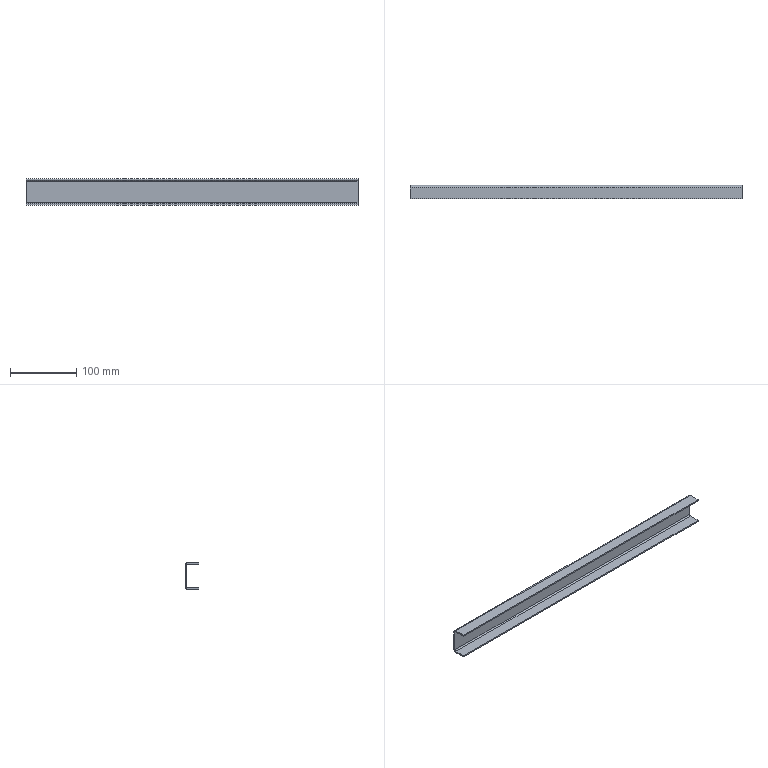Component | SolidWorks | DoorAssembly-1_DoorStiffener-1 | 1 solid | 22 faces | box 500 x 20 x 40 mm | volume 73425 mm3 | plane 18 | cylinder 4 | commonest cylinder face diameters 8 x2 4 x2 | material Plain Carbon Steel
STEP:
#1=COLOUR_RGB('',0.7922,0.8196,0.9333);
#2=FILL_AREA_STYLE_COLOUR('',#1);
#3=FILL_AREA_STYLE('',(#2));
#4=SURFACE_STYLE_FILL_AREA(#3);
#5=SURFACE_SIDE_STYLE('',(#4));
#6=SURFACE_STYLE_USAGE(.BOTH.,#5);
#7=PRESENTATION_STYLE_ASSIGNMENT((#6));
#8=CARTESIAN_POINT('',(21.724,-0.5689,59.724));
#9=VERTEX_POINT('',#8);
#10=CARTESIAN_POINT('',(21.724,-0.6477,59.724));
#11=VERTEX_POINT('',#10);
#12=CARTESIAN_POINT('',(21.724,-0.5689,59.724));
#13=DIRECTION('',(-0.,-1.,0.));
#14=VECTOR('',#13,39.37);
#15=LINE('',#12,#14);
#16=EDGE_CURVE('',#9,#11,#15,.T.);
#17=ORIENTED_EDGE('',*,*,#16,.F.);
#18=CARTESIAN_POINT('',(21.724,-0.7264,59.566));
#19=VERTEX_POINT('',#18);
#20=CARTESIAN_POINT('',(21.724,-0.7264,59.724));
#21=DIRECTION('',(1.,-0.,-0.));
#22=DIRECTION('',(0.,0.,1.));
#23=AXIS2_PLACEMENT_3D('',#20,#21,#22);
#24=CIRCLE('',#23,0.1575);
#25=EDGE_CURVE('',#19,#9,#24,.T.);
#26=ORIENTED_EDGE('',*,*,#25,.F.);
#27=CARTESIAN_POINT('',(21.724,-0.7264,59.645));
#28=VERTEX_POINT('',#27);
#29=CARTESIAN_POINT('',(21.724,-0.7264,59.645));
#30=DIRECTION('',(-0.,-0.,-1.));
#31=VECTOR('',#30,39.37);
#32=LINE('',#29,#31);
#33=EDGE_CURVE('',#28,#19,#32,.T.);
#34=ORIENTED_EDGE('',*,*,#33,.F.);
#35=CARTESIAN_POINT('',(21.724,-0.7264,59.724));
#36=DIRECTION('',(1.,-0.,-0.));
#37=DIRECTION('',(0.,0.,1.));
#38=AXIS2_PLACEMENT_3D('',#35,#36,#37);
#39=CIRCLE('',#38,0.07874);
#40=EDGE_CURVE('',#28,#11,#39,.T.);
#41=ORIENTED_EDGE('',*,*,#40,.T.);
#42=EDGE_LOOP('',(#17,#26,#34,#41));
#43=FACE_OUTER_BOUND('',#42,.T.);
#44=CARTESIAN_POINT('',(21.724,-0.5689,59.724));
#45=DIRECTION('',(-1.,0.,0.));
#46=DIRECTION('',(0.,0.,1.));
#47=AXIS2_PLACEMENT_3D('',#44,#45,#46);
#48=PLANE('',#47);
#49=ADVANCED_FACE('',(#43),#48,.T.);
#50=CARTESIAN_POINT('',(21.724,-0.5689,60.983));
#51=VERTEX_POINT('',#50);
#52=CARTESIAN_POINT('',(21.724,-0.5689,59.566));
#53=DIRECTION('',(0.,0.,1.));
#54=VECTOR('',#53,39.37);
#55=LINE('',#52,#54);
#56=EDGE_CURVE('',#9,#51,#55,.T.);
#57=ORIENTED_EDGE('',*,*,#56,.F.);
#58=ORIENTED_EDGE('',*,*,#16,.T.);
#59=CARTESIAN_POINT('',(21.724,-0.6477,60.983));
#60=VERTEX_POINT('',#59);
#61=CARTESIAN_POINT('',(21.724,-0.6477,59.566));
#62=DIRECTION('',(0.,0.,1.));
#63=VECTOR('',#62,39.37);
#64=LINE('',#61,#63);
#65=EDGE_CURVE('',#11,#60,#64,.T.);
#66=ORIENTED_EDGE('',*,*,#65,.T.);
#67=CARTESIAN_POINT('',(21.724,-0.6477,60.983));
#68=DIRECTION('',(0.,1.,-0.));
#69=VECTOR('',#68,39.37);
#70=LINE('',#67,#69);
#71=EDGE_CURVE('',#60,#51,#70,.T.);
#72=ORIENTED_EDGE('',*,*,#71,.T.);
#73=EDGE_LOOP('',(#57,#58,#66,#72));
#74=FACE_OUTER_BOUND('',#73,.T.);
#75=CARTESIAN_POINT('',(21.724,-0.7264,59.645));
#76=DIRECTION('',(-1.,0.,0.));
#77=DIRECTION('',(0.,0.,1.));
#78=AXIS2_PLACEMENT_3D('',#75,#76,#77);
#79=PLANE('',#78);
#80=ADVANCED_FACE('',(#74),#79,.T.);
#81=CARTESIAN_POINT('',(41.409,-0.7264,59.566));
#82=VERTEX_POINT('',#81);
#83=CARTESIAN_POINT('',(41.409,-0.7264,59.645));
#84=VERTEX_POINT('',#83);
#85=CARTESIAN_POINT('',(41.409,-0.7264,59.566));
#86=DIRECTION('',(0.,0.,1.));
#87=VECTOR('',#86,39.37);
#88=LINE('',#85,#87);
#89=EDGE_CURVE('',#82,#84,#88,.T.);
#90=ORIENTED_EDGE('',*,*,#89,.F.);
#91=CARTESIAN_POINT('',(41.409,-0.5689,59.724));
#92=VERTEX_POINT('',#91);
#93=CARTESIAN_POINT('',(41.409,-0.7264,59.724));
#94=DIRECTION('',(1.,-0.,-0.));
#95=DIRECTION('',(0.,0.,1.));
#96=AXIS2_PLACEMENT_3D('',#93,#94,#95);
#97=CIRCLE('',#96,0.1575);
#98=EDGE_CURVE('',#82,#92,#97,.T.);
#99=ORIENTED_EDGE('',*,*,#98,.T.);
#100=CARTESIAN_POINT('',(41.409,-0.6477,59.724));
#101=VERTEX_POINT('',#100);
#102=CARTESIAN_POINT('',(41.409,-0.6477,59.724));
#103=DIRECTION('',(0.,1.,-0.));
#104=VECTOR('',#103,39.37);
#105=LINE('',#102,#104);
#106=EDGE_CURVE('',#101,#92,#105,.T.);
#107=ORIENTED_EDGE('',*,*,#106,.F.);
#108=CARTESIAN_POINT('',(41.409,-0.7264,59.724));
#109=DIRECTION('',(1.,-0.,-0.));
#110=DIRECTION('',(0.,0.,1.));
#111=AXIS2_PLACEMENT_3D('',#108,#109,#110);
#112=CIRCLE('',#111,0.07874);
#113=EDGE_CURVE('',#84,#101,#112,.T.);
#114=ORIENTED_EDGE('',*,*,#113,.F.);
#115=EDGE_LOOP('',(#90,#99,#107,#114));
#116=FACE_OUTER_BOUND('',#115,.T.);
#117=CARTESIAN_POINT('',(41.409,-0.7264,59.566));
#118=DIRECTION('',(1.,-0.,-0.));
#119=DIRECTION('',(-0.,-0.,-1.));
#120=AXIS2_PLACEMENT_3D('',#117,#118,#119);
#121=PLANE('',#120);
#122=ADVANCED_FACE('',(#116),#121,.T.);
#123=CARTESIAN_POINT('',(41.409,-1.356,59.566));
#124=VERTEX_POINT('',#123);
#125=CARTESIAN_POINT('',(41.409,-1.356,59.566));
#126=DIRECTION('',(0.,1.,-0.));
#127=VECTOR('',#126,39.37);
#128=LINE('',#125,#127);
#129=EDGE_CURVE('',#124,#82,#128,.T.);
#130=ORIENTED_EDGE('',*,*,#129,.T.);
#131=ORIENTED_EDGE('',*,*,#89,.T.);
#132=CARTESIAN_POINT('',(41.409,-1.356,59.645));
#133=VERTEX_POINT('',#132);
#134=CARTESIAN_POINT('',(41.409,-1.356,59.645));
#135=DIRECTION('',(0.,1.,-0.));
#136=VECTOR('',#135,39.37);
#137=LINE('',#134,#136);
#138=EDGE_CURVE('',#133,#84,#137,.T.);
#139=ORIENTED_EDGE('',*,*,#138,.F.);
#140=CARTESIAN_POINT('',(41.409,-1.356,59.645));
#141=DIRECTION('',(-0.,-0.,-1.));
#142=VECTOR('',#141,39.37);
#143=LINE('',#140,#142);
#144=EDGE_CURVE('',#133,#124,#143,.T.);
#145=ORIENTED_EDGE('',*,*,#144,.T.);
#146=EDGE_LOOP('',(#130,#131,#139,#145));
#147=FACE_OUTER_BOUND('',#146,.T.);
#148=CARTESIAN_POINT('',(41.409,-0.6477,59.724));
#149=DIRECTION('',(1.,-0.,-0.));
#150=DIRECTION('',(-0.,-0.,-1.));
#151=AXIS2_PLACEMENT_3D('',#148,#149,#150);
#152=PLANE('',#151);
#153=ADVANCED_FACE('',(#147),#152,.T.);
#154=CARTESIAN_POINT('',(21.724,-0.7264,61.141));
#155=VERTEX_POINT('',#154);
#156=CARTESIAN_POINT('',(21.724,-0.7264,61.062));
#157=VERTEX_POINT('',#156);
#158=CARTESIAN_POINT('',(21.724,-0.7264,61.141));
#159=DIRECTION('',(-0.,-0.,-1.));
#160=VECTOR('',#159,39.37);
#161=LINE('',#158,#160);
#162=EDGE_CURVE('',#155,#157,#161,.T.);
#163=ORIENTED_EDGE('',*,*,#162,.F.);
#164=CARTESIAN_POINT('',(21.724,-0.7264,60.983));
#165=DIRECTION('',(1.,-0.,-0.));
#166=DIRECTION('',(0.,0.,1.));
#167=AXIS2_PLACEMENT_3D('',#164,#165,#166);
#168=CIRCLE('',#167,0.1575);
#169=EDGE_CURVE('',#51,#155,#168,.T.);
#170=ORIENTED_EDGE('',*,*,#169,.F.);
#171=ORIENTED_EDGE('',*,*,#71,.F.);
#172=CARTESIAN_POINT('',(21.724,-0.7264,60.983));
#173=DIRECTION('',(1.,-0.,-0.));
#174=DIRECTION('',(0.,0.,1.));
#175=AXIS2_PLACEMENT_3D('',#172,#173,#174);
#176=CIRCLE('',#175,0.07874);
#177=EDGE_CURVE('',#60,#157,#176,.T.);
#178=ORIENTED_EDGE('',*,*,#177,.T.);
#179=EDGE_LOOP('',(#163,#170,#171,#178));
#180=FACE_OUTER_BOUND('',#179,.T.);
#181=CARTESIAN_POINT('',(21.724,-0.7264,61.141));
#182=DIRECTION('',(-1.,0.,0.));
#183=DIRECTION('',(0.,0.,1.));
#184=AXIS2_PLACEMENT_3D('',#181,#182,#183);
#185=PLANE('',#184);
#186=ADVANCED_FACE('',(#180),#185,.T.);
#187=CARTESIAN_POINT('',(21.724,-1.356,61.141));
#188=VERTEX_POINT('',#187);
#189=CARTESIAN_POINT('',(21.724,-0.5689,61.141));
#190=DIRECTION('',(-0.,-1.,0.));
#191=VECTOR('',#190,39.37);
#192=LINE('',#189,#191);
#193=EDGE_CURVE('',#155,#188,#192,.T.);
#194=ORIENTED_EDGE('',*,*,#193,.F.);
#195=ORIENTED_EDGE('',*,*,#162,.T.);
#196=CARTESIAN_POINT('',(21.724,-1.356,61.062));
#197=VERTEX_POINT('',#196);
#198=CARTESIAN_POINT('',(21.724,-0.5689,61.062));
#199=DIRECTION('',(-0.,-1.,0.));
#200=VECTOR('',#199,39.37);
#201=LINE('',#198,#200);
#202=EDGE_CURVE('',#157,#197,#201,.T.);
#203=ORIENTED_EDGE('',*,*,#202,.T.);
#204=CARTESIAN_POINT('',(21.724,-1.356,61.141));
#205=DIRECTION('',(-0.,-0.,-1.));
#206=VECTOR('',#205,39.37);
#207=LINE('',#204,#206);
#208=EDGE_CURVE('',#188,#197,#207,.T.);
#209=ORIENTED_EDGE('',*,*,#208,.F.);
#210=EDGE_LOOP('',(#194,#195,#203,#209));
#211=FACE_OUTER_BOUND('',#210,.T.);
#212=CARTESIAN_POINT('',(21.724,-0.6477,60.983));
#213=DIRECTION('',(-1.,0.,0.));
#214=DIRECTION('',(0.,0.,1.));
#215=AXIS2_PLACEMENT_3D('',#212,#213,#214);
#216=PLANE('',#215);
#217=ADVANCED_FACE('',(#211),#216,.T.);
#218=CARTESIAN_POINT('',(41.409,-0.5689,60.983));
#219=VERTEX_POINT('',#218);
#220=CARTESIAN_POINT('',(41.409,-0.6477,60.983));
#221=VERTEX_POINT('',#220);
#222=CARTESIAN_POINT('',(41.409,-0.5689,60.983));
#223=DIRECTION('',(-0.,-1.,0.));
#224=VECTOR('',#223,39.37);
#225=LINE('',#222,#224);
#226=EDGE_CURVE('',#219,#221,#225,.T.);
#227=ORIENTED_EDGE('',*,*,#226,.F.);
#228=CARTESIAN_POINT('',(41.409,-0.7264,61.141));
#229=VERTEX_POINT('',#228);
#230=CARTESIAN_POINT('',(41.409,-0.7264,60.983));
#231=DIRECTION('',(1.,-0.,-0.));
#232=DIRECTION('',(0.,0.,1.));
#233=AXIS2_PLACEMENT_3D('',#230,#231,#232);
#234=CIRCLE('',#233,0.1575);
#235=EDGE_CURVE('',#219,#229,#234,.T.);
#236=ORIENTED_EDGE('',*,*,#235,.T.);
#237=CARTESIAN_POINT('',(41.409,-0.7264,61.062));
#238=VERTEX_POINT('',#237);
#239=CARTESIAN_POINT('',(41.409,-0.7264,61.062));
#240=DIRECTION('',(0.,0.,1.));
#241=VECTOR('',#240,39.37);
#242=LINE('',#239,#241);
#243=EDGE_CURVE('',#238,#229,#242,.T.);
#244=ORIENTED_EDGE('',*,*,#243,.F.);
#245=CARTESIAN_POINT('',(41.409,-0.7264,60.983));
#246=DIRECTION('',(1.,-0.,-0.));
#247=DIRECTION('',(0.,0.,1.));
#248=AXIS2_PLACEMENT_3D('',#245,#246,#247);
#249=CIRCLE('',#248,0.07874);
#250=EDGE_CURVE('',#221,#238,#249,.T.);
#251=ORIENTED_EDGE('',*,*,#250,.F.);
#252=EDGE_LOOP('',(#227,#236,#244,#251));
#253=FACE_OUTER_BOUND('',#252,.T.);
#254=CARTESIAN_POINT('',(41.409,-0.5689,60.983));
#255=DIRECTION('',(1.,-0.,-0.));
#256=DIRECTION('',(-0.,-0.,-1.));
#257=AXIS2_PLACEMENT_3D('',#254,#255,#256);
#258=PLANE('',#257);
#259=ADVANCED_FACE('',(#253),#258,.T.);
#260=CARTESIAN_POINT('',(41.409,-0.5689,59.566));
#261=DIRECTION('',(0.,0.,1.));
#262=VECTOR('',#261,39.37);
#263=LINE('',#260,#262);
#264=EDGE_CURVE('',#92,#219,#263,.T.);
#265=ORIENTED_EDGE('',*,*,#264,.T.);
#266=ORIENTED_EDGE('',*,*,#226,.T.);
#267=CARTESIAN_POINT('',(41.409,-0.6477,59.566));
#268=DIRECTION('',(0.,0.,1.));
#269=VECTOR('',#268,39.37);
#270=LINE('',#267,#269);
#271=EDGE_CURVE('',#101,#221,#270,.T.);
#272=ORIENTED_EDGE('',*,*,#271,.F.);
#273=ORIENTED_EDGE('',*,*,#106,.T.);
#274=EDGE_LOOP('',(#265,#266,#272,#273));
#275=FACE_OUTER_BOUND('',#274,.T.);
#276=CARTESIAN_POINT('',(41.409,-0.7264,61.062));
#277=DIRECTION('',(1.,-0.,-0.));
#278=DIRECTION('',(-0.,-0.,-1.));
#279=AXIS2_PLACEMENT_3D('',#276,#277,#278);
#280=PLANE('',#279);
#281=ADVANCED_FACE('',(#275),#280,.T.);
#282=CARTESIAN_POINT('',(41.409,-1.356,61.062));
#283=VERTEX_POINT('',#282);
#284=CARTESIAN_POINT('',(41.409,-0.5689,61.062));
#285=DIRECTION('',(-0.,-1.,0.));
#286=VECTOR('',#285,39.37);
#287=LINE('',#284,#286);
#288=EDGE_CURVE('',#238,#283,#287,.T.);
#289=ORIENTED_EDGE('',*,*,#288,.T.);
#290=CARTESIAN_POINT('',(21.724,-1.356,61.062));
#291=DIRECTION('',(1.,-0.,-0.));
#292=VECTOR('',#291,39.37);
#293=LINE('',#290,#292);
#294=EDGE_CURVE('',#197,#283,#293,.T.);
#295=ORIENTED_EDGE('',*,*,#294,.F.);
#296=ORIENTED_EDGE('',*,*,#202,.F.);
#297=CARTESIAN_POINT('',(21.724,-0.7264,61.062));
#298=DIRECTION('',(1.,-0.,-0.));
#299=VECTOR('',#298,39.37);
#300=LINE('',#297,#299);
#301=EDGE_CURVE('',#157,#238,#300,.T.);
#302=ORIENTED_EDGE('',*,*,#301,.T.);
#303=EDGE_LOOP('',(#289,#295,#296,#302));
#304=FACE_OUTER_BOUND('',#303,.T.);
#305=CARTESIAN_POINT('',(21.724,-0.5689,61.062));
#306=DIRECTION('',(0.,0.,1.));
#307=DIRECTION('',(1.,-0.,-0.));
#308=AXIS2_PLACEMENT_3D('',#305,#306,#307);
#309=PLANE('',#308);
#310=ADVANCED_FACE('',(#304),#309,.F.);
#311=CARTESIAN_POINT('',(41.409,-1.356,61.141));
#312=VERTEX_POINT('',#311);
#313=CARTESIAN_POINT('',(41.409,-1.356,61.141));
#314=DIRECTION('',(-0.,-0.,-1.));
#315=VECTOR('',#314,39.37);
#316=LINE('',#313,#315);
#317=EDGE_CURVE('',#312,#283,#316,.T.);
#318=ORIENTED_EDGE('',*,*,#317,.F.);
#319=CARTESIAN_POINT('',(21.724,-1.356,61.141));
#320=DIRECTION('',(1.,-0.,-0.));
#321=VECTOR('',#320,39.37);
#322=LINE('',#319,#321);
#323=EDGE_CURVE('',#188,#312,#322,.T.);
#324=ORIENTED_EDGE('',*,*,#323,.F.);
#325=ORIENTED_EDGE('',*,*,#208,.T.);
#326=ORIENTED_EDGE('',*,*,#294,.T.);
#327=EDGE_LOOP('',(#318,#324,#325,#326));
#328=FACE_OUTER_BOUND('',#327,.T.);
#329=CARTESIAN_POINT('',(21.724,-1.356,61.141));
#330=DIRECTION('',(-0.,-1.,0.));
#331=DIRECTION('',(1.,-0.,-0.));
#332=AXIS2_PLACEMENT_3D('',#329,#330,#331);
#333=PLANE('',#332);
#334=ADVANCED_FACE('',(#328),#333,.T.);
#335=CARTESIAN_POINT('',(41.409,-0.5689,61.141));
#336=DIRECTION('',(-0.,-1.,0.));
#337=VECTOR('',#336,39.37);
#338=LINE('',#335,#337);
#339=EDGE_CURVE('',#229,#312,#338,.T.);
#340=ORIENTED_EDGE('',*,*,#339,.F.);
#341=CARTESIAN_POINT('',(21.724,-0.7264,61.141));
#342=DIRECTION('',(1.,-0.,-0.));
#343=VECTOR('',#342,39.37);
#344=LINE('',#341,#343);
#345=EDGE_CURVE('',#155,#229,#344,.T.);
#346=ORIENTED_EDGE('',*,*,#345,.F.);
#347=ORIENTED_EDGE('',*,*,#193,.T.);
#348=ORIENTED_EDGE('',*,*,#323,.T.);
#349=EDGE_LOOP('',(#340,#346,#347,#348));
#350=FACE_OUTER_BOUND('',#349,.T.);
#351=CARTESIAN_POINT('',(21.724,-0.5689,61.141));
#352=DIRECTION('',(0.,0.,1.));
#353=DIRECTION('',(1.,-0.,-0.));
#354=AXIS2_PLACEMENT_3D('',#351,#352,#353);
#355=PLANE('',#354);
#356=ADVANCED_FACE('',(#350),#355,.T.);
#357=ORIENTED_EDGE('',*,*,#235,.F.);
#358=CARTESIAN_POINT('',(21.724,-0.5689,60.983));
#359=DIRECTION('',(1.,-0.,-0.));
#360=VECTOR('',#359,39.37);
#361=LINE('',#358,#360);
#362=EDGE_CURVE('',#51,#219,#361,.T.);
#363=ORIENTED_EDGE('',*,*,#362,.F.);
#364=ORIENTED_EDGE('',*,*,#169,.T.);
#365=ORIENTED_EDGE('',*,*,#345,.T.);
#366=EDGE_LOOP('',(#357,#363,#364,#365));
#367=FACE_OUTER_BOUND('',#366,.T.);
#368=CARTESIAN_POINT('',(21.724,-0.7264,60.983));
#369=DIRECTION('',(1.,-0.,-0.));
#370=DIRECTION('',(0.,-0.,-1.));
#371=AXIS2_PLACEMENT_3D('',#368,#369,#370);
#372=CYLINDRICAL_SURFACE('',#371,0.1575);
#373=ADVANCED_FACE('',(#367),#372,.T.);
#374=ORIENTED_EDGE('',*,*,#264,.F.);
#375=CARTESIAN_POINT('',(21.724,-0.5689,59.724));
#376=DIRECTION('',(1.,-0.,-0.));
#377=VECTOR('',#376,39.37);
#378=LINE('',#375,#377);
#379=EDGE_CURVE('',#9,#92,#378,.T.);
#380=ORIENTED_EDGE('',*,*,#379,.F.);
#381=ORIENTED_EDGE('',*,*,#56,.T.);
#382=ORIENTED_EDGE('',*,*,#362,.T.);
#383=EDGE_LOOP('',(#374,#380,#381,#382));
#384=FACE_OUTER_BOUND('',#383,.T.);
#385=CARTESIAN_POINT('',(21.724,-0.5689,59.566));
#386=DIRECTION('',(0.,1.,-0.));
#387=DIRECTION('',(-1.,0.,0.));
#388=AXIS2_PLACEMENT_3D('',#385,#386,#387);
#389=PLANE('',#388);
#390=ADVANCED_FACE('',(#384),#389,.T.);
#391=ORIENTED_EDGE('',*,*,#98,.F.);
#392=CARTESIAN_POINT('',(21.724,-0.7264,59.566));
#393=DIRECTION('',(1.,-0.,-0.));
#394=VECTOR('',#393,39.37);
#395=LINE('',#392,#394);
#396=EDGE_CURVE('',#19,#82,#395,.T.);
#397=ORIENTED_EDGE('',*,*,#396,.F.);
#398=ORIENTED_EDGE('',*,*,#25,.T.);
#399=ORIENTED_EDGE('',*,*,#379,.T.);
#400=EDGE_LOOP('',(#391,#397,#398,#399));
#401=FACE_OUTER_BOUND('',#400,.T.);
#402=CARTESIAN_POINT('',(21.724,-0.7264,59.724));
#403=DIRECTION('',(1.,-0.,-0.));
#404=DIRECTION('',(0.,-0.,-1.));
#405=AXIS2_PLACEMENT_3D('',#402,#403,#404);
#406=CYLINDRICAL_SURFACE('',#405,0.1575);
#407=ADVANCED_FACE('',(#401),#406,.T.);
#408=ORIENTED_EDGE('',*,*,#129,.F.);
#409=CARTESIAN_POINT('',(21.724,-1.356,59.566));
#410=VERTEX_POINT('',#409);
#411=CARTESIAN_POINT('',(21.724,-1.356,59.566));
#412=DIRECTION('',(1.,-0.,-0.));
#413=VECTOR('',#412,39.37);
#414=LINE('',#411,#413);
#415=EDGE_CURVE('',#410,#124,#414,.T.);
#416=ORIENTED_EDGE('',*,*,#415,.F.);
#417=CARTESIAN_POINT('',(21.724,-1.356,59.566));
#418=DIRECTION('',(0.,1.,-0.));
#419=VECTOR('',#418,39.37);
#420=LINE('',#417,#419);
#421=EDGE_CURVE('',#410,#19,#420,.T.);
#422=ORIENTED_EDGE('',*,*,#421,.T.);
#423=ORIENTED_EDGE('',*,*,#396,.T.);
#424=EDGE_LOOP('',(#408,#416,#422,#423));
#425=FACE_OUTER_BOUND('',#424,.T.);
#426=CARTESIAN_POINT('',(21.724,-1.356,59.566));
#427=DIRECTION('',(-0.,-0.,-1.));
#428=DIRECTION('',(-1.,0.,0.));
#429=AXIS2_PLACEMENT_3D('',#426,#427,#428);
#430=PLANE('',#429);
#431=ADVANCED_FACE('',(#425),#430,.T.);
#432=ORIENTED_EDGE('',*,*,#144,.F.);
#433=CARTESIAN_POINT('',(21.724,-1.356,59.645));
#434=VERTEX_POINT('',#433);
#435=CARTESIAN_POINT('',(21.724,-1.356,59.645));
#436=DIRECTION('',(1.,-0.,-0.));
#437=VECTOR('',#436,39.37);
#438=LINE('',#435,#437);
#439=EDGE_CURVE('',#434,#133,#438,.T.);
#440=ORIENTED_EDGE('',*,*,#439,.F.);
#441=CARTESIAN_POINT('',(21.724,-1.356,59.645));
#442=DIRECTION('',(-0.,-0.,-1.));
#443=VECTOR('',#442,39.37);
#444=LINE('',#441,#443);
#445=EDGE_CURVE('',#434,#410,#444,.T.);
#446=ORIENTED_EDGE('',*,*,#445,.T.);
#447=ORIENTED_EDGE('',*,*,#415,.T.);
#448=EDGE_LOOP('',(#432,#440,#446,#447));
#449=FACE_OUTER_BOUND('',#448,.T.);
#450=CARTESIAN_POINT('',(21.724,-1.356,59.645));
#451=DIRECTION('',(-0.,-1.,0.));
#452=DIRECTION('',(1.,-0.,-0.));
#453=AXIS2_PLACEMENT_3D('',#450,#451,#452);
#454=PLANE('',#453);
#455=ADVANCED_FACE('',(#449),#454,.T.);
#456=ORIENTED_EDGE('',*,*,#138,.T.);
#457=CARTESIAN_POINT('',(21.724,-0.7264,59.645));
#458=DIRECTION('',(1.,-0.,-0.));
#459=VECTOR('',#458,39.37);
#460=LINE('',#457,#459);
#461=EDGE_CURVE('',#28,#84,#460,.T.);
#462=ORIENTED_EDGE('',*,*,#461,.F.);
#463=CARTESIAN_POINT('',(21.724,-1.356,59.645));
#464=DIRECTION('',(0.,1.,-0.));
#465=VECTOR('',#464,39.37);
#466=LINE('',#463,#465);
#467=EDGE_CURVE('',#434,#28,#466,.T.);
#468=ORIENTED_EDGE('',*,*,#467,.F.);
#469=ORIENTED_EDGE('',*,*,#439,.T.);
#470=EDGE_LOOP('',(#456,#462,#468,#469));
#471=FACE_OUTER_BOUND('',#470,.T.);
#472=CARTESIAN_POINT('',(21.724,-1.356,59.645));
#473=DIRECTION('',(-0.,-0.,-1.));
#474=DIRECTION('',(-1.,0.,0.));
#475=AXIS2_PLACEMENT_3D('',#472,#473,#474);
#476=PLANE('',#475);
#477=ADVANCED_FACE('',(#471),#476,.F.);
#478=ORIENTED_EDGE('',*,*,#113,.T.);
#479=CARTESIAN_POINT('',(21.724,-0.6477,59.724));
#480=DIRECTION('',(1.,-0.,-0.));
#481=VECTOR('',#480,39.37);
#482=LINE('',#479,#481);
#483=EDGE_CURVE('',#11,#101,#482,.T.);
#484=ORIENTED_EDGE('',*,*,#483,.F.);
#485=ORIENTED_EDGE('',*,*,#40,.F.);
#486=ORIENTED_EDGE('',*,*,#461,.T.);
#487=EDGE_LOOP('',(#478,#484,#485,#486));
#488=FACE_OUTER_BOUND('',#487,.T.);
#489=CARTESIAN_POINT('',(21.724,-0.7264,59.724));
#490=DIRECTION('',(1.,-0.,-0.));
#491=DIRECTION('',(0.,-0.,-1.));
#492=AXIS2_PLACEMENT_3D('',#489,#490,#491);
#493=CYLINDRICAL_SURFACE('',#492,0.07874);
#494=ADVANCED_FACE('',(#488),#493,.F.);
#495=ORIENTED_EDGE('',*,*,#271,.T.);
#496=CARTESIAN_POINT('',(21.724,-0.6477,60.983));
#497=DIRECTION('',(1.,-0.,-0.));
#498=VECTOR('',#497,39.37);
#499=LINE('',#496,#498);
#500=EDGE_CURVE('',#60,#221,#499,.T.);
#501=ORIENTED_EDGE('',*,*,#500,.F.);
#502=ORIENTED_EDGE('',*,*,#65,.F.);
#503=ORIENTED_EDGE('',*,*,#483,.T.);
#504=EDGE_LOOP('',(#495,#501,#502,#503));
#505=FACE_OUTER_BOUND('',#504,.T.);
#506=CARTESIAN_POINT('',(21.724,-0.6477,59.566));
#507=DIRECTION('',(0.,1.,-0.));
#508=DIRECTION('',(-1.,0.,0.));
#509=AXIS2_PLACEMENT_3D('',#506,#507,#508);
#510=PLANE('',#509);
#511=ADVANCED_FACE('',(#505),#510,.F.);
#512=ORIENTED_EDGE('',*,*,#250,.T.);
#513=ORIENTED_EDGE('',*,*,#301,.F.);
#514=ORIENTED_EDGE('',*,*,#177,.F.);
#515=ORIENTED_EDGE('',*,*,#500,.T.);
#516=EDGE_LOOP('',(#512,#513,#514,#515));
#517=FACE_OUTER_BOUND('',#516,.T.);
#518=CARTESIAN_POINT('',(21.724,-0.7264,60.983));
#519=DIRECTION('',(1.,-0.,-0.));
#520=DIRECTION('',(0.,-0.,-1.));
#521=AXIS2_PLACEMENT_3D('',#518,#519,#520);
#522=CYLINDRICAL_SURFACE('',#521,0.07874);
#523=ADVANCED_FACE('',(#517),#522,.F.);
#524=ORIENTED_EDGE('',*,*,#467,.T.);
#525=ORIENTED_EDGE('',*,*,#33,.T.);
#526=ORIENTED_EDGE('',*,*,#421,.F.);
#527=ORIENTED_EDGE('',*,*,#445,.F.);
#528=EDGE_LOOP('',(#524,#525,#526,#527));
#529=FACE_OUTER_BOUND('',#528,.T.);
#530=CARTESIAN_POINT('',(21.724,-0.7264,60.983));
#531=DIRECTION('',(-1.,0.,0.));
#532=DIRECTION('',(0.,0.,1.));
#533=AXIS2_PLACEMENT_3D('',#530,#531,#532);
#534=PLANE('',#533);
#535=ADVANCED_FACE('',(#529),#534,.T.);
#536=ORIENTED_EDGE('',*,*,#288,.F.);
#537=ORIENTED_EDGE('',*,*,#243,.T.);
#538=ORIENTED_EDGE('',*,*,#339,.T.);
#539=ORIENTED_EDGE('',*,*,#317,.T.);
#540=EDGE_LOOP('',(#536,#537,#538,#539));
#541=FACE_OUTER_BOUND('',#540,.T.);
#542=CARTESIAN_POINT('',(41.409,-0.7264,60.983));
#543=DIRECTION('',(-1.,0.,0.));
#544=DIRECTION('',(0.,0.,1.));
#545=AXIS2_PLACEMENT_3D('',#542,#543,#544);
#546=PLANE('',#545);
#547=ADVANCED_FACE('',(#541),#546,.F.);
#548=CLOSED_SHELL('',(#49,#80,#122,#153,#186,#217,#259,#281,#310,#334,#356,#373,#390,#407,#431,#455,#477,#494,#511,#523,#535,#547));
#549=MANIFOLD_SOLID_BREP('',#548);
#550=STYLED_ITEM('',(#7),#549);
#551=(LENGTH_UNIT()NAMED_UNIT(*)SI_UNIT($,.METRE.));
#552=LENGTH_MEASURE_WITH_UNIT(LENGTH_MEASURE(0.0254),#551);
#553=DIMENSIONAL_EXPONENTS(1.,0.,0.,0.,0.,0.,0.);
#554=(CONVERSION_BASED_UNIT('',#552)LENGTH_UNIT()NAMED_UNIT(#553));
#555=UNCERTAINTY_MEASURE_WITH_UNIT(LENGTH_MEASURE(0.00001),#554,'','');
#556=(NAMED_UNIT(*)PLANE_ANGLE_UNIT()SI_UNIT($,.RADIAN.));
#557=(NAMED_UNIT(*)SI_UNIT($,.STERADIAN.)SOLID_ANGLE_UNIT());
#558=(GEOMETRIC_REPRESENTATION_CONTEXT(3)GLOBAL_UNCERTAINTY_ASSIGNED_CONTEXT((#555))GLOBAL_UNIT_ASSIGNED_CONTEXT((#554,#556,#557))REPRESENTATION_CONTEXT('',''));
#559=MECHANICAL_DESIGN_GEOMETRIC_PRESENTATION_REPRESENTATION('',(#550),#558);
#560=PRESENTATION_LAYER_ASSIGNMENT('','',(#550));
#561=CARTESIAN_POINT('',(0.,0.,0.));
#562=DIRECTION('',(0.,0.,1.));
#563=DIRECTION('',(1.,0.,0.));
#564=AXIS2_PLACEMENT_3D('',#561,#562,#563);
#565=(LENGTH_UNIT()NAMED_UNIT(*)SI_UNIT($,.METRE.));
#566=LENGTH_MEASURE_WITH_UNIT(LENGTH_MEASURE(0.0254),#565);
#567=DIMENSIONAL_EXPONENTS(1.,0.,0.,0.,0.,0.,0.);
#568=(CONVERSION_BASED_UNIT('',#566)LENGTH_UNIT()NAMED_UNIT(#567));
#569=UNCERTAINTY_MEASURE_WITH_UNIT(LENGTH_MEASURE(0.00001),#568,'','');
#570=(NAMED_UNIT(*)PLANE_ANGLE_UNIT()SI_UNIT($,.RADIAN.));
#571=(NAMED_UNIT(*)SI_UNIT($,.STERADIAN.)SOLID_ANGLE_UNIT());
#572=(GEOMETRIC_REPRESENTATION_CONTEXT(3)GLOBAL_UNCERTAINTY_ASSIGNED_CONTEXT((#569))GLOBAL_UNIT_ASSIGNED_CONTEXT((#568,#570,#571))REPRESENTATION_CONTEXT('',''));
#573=ADVANCED_BREP_SHAPE_REPRESENTATION('',(#549,#564),#572);